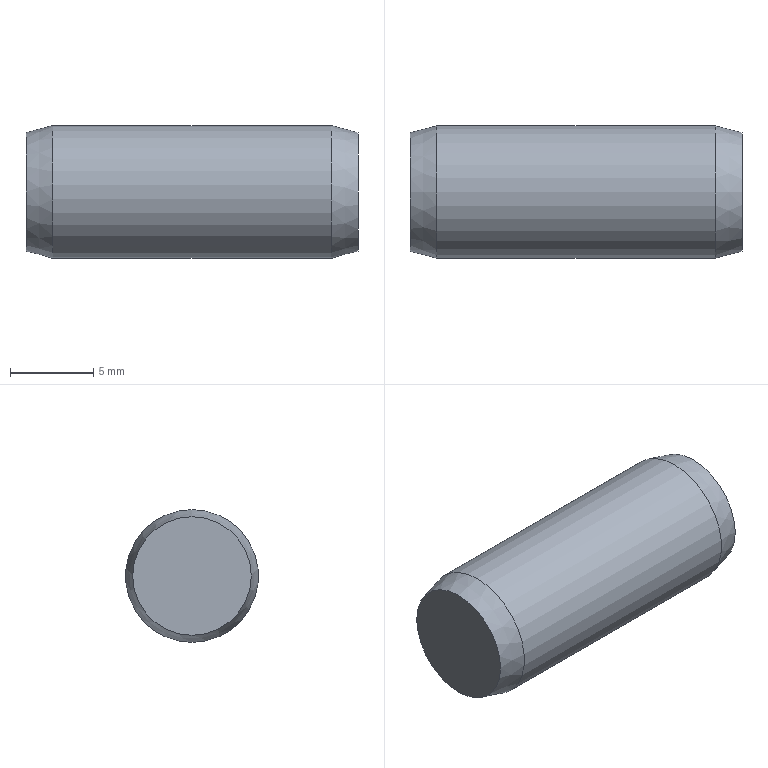Component | NX | GB-T119_1-2000_8X20_2 | 1 solid | 5 faces | box 20 x 8 x 8 mm | volume 989 mm3 | plane 2 | cone 2 | cylinder 1 | commonest cylinder face diameters 8 x1
STEP:
#1=CARTESIAN_POINT('',(0.,0.,0.));
#2=DIRECTION('',(0.,0.,1.));
#3=DIRECTION('',(1.,0.,0.));
#4=AXIS2_PLACEMENT_3D('',#1,#2,#3);
#5=CARTESIAN_POINT('',(-7.89,-28.599,-193.805));
#6=VERTEX_POINT('',#5);
#7=CARTESIAN_POINT('',(-7.89,-28.599,-197.377));
#8=DIRECTION('',(-1.,0.,0.));
#9=DIRECTION('',(0.,0.,1.));
#10=AXIS2_PLACEMENT_3D('',#7,#8,#9);
#11=CIRCLE('',#10,3.571);
#12=CARTESIAN_POINT('',(-7.89,-28.599,-197.377));
#13=DIRECTION('',(-1.,0.,0.));
#14=DIRECTION('',(0.,0.,1.));
#15=AXIS2_PLACEMENT_3D('',#12,#13,#14);
#16=PLANE('',#15);
#17=CARTESIAN_POINT('',(0.,0.));
#18=DIRECTION('',(1.,0.));
#19=AXIS2_PLACEMENT_2D('',#17,#18);
#20=CIRCLE('',#19,3.571);
#21=(GEOMETRIC_REPRESENTATION_CONTEXT(2)PARAMETRIC_REPRESENTATION_CONTEXT()REPRESENTATION_CONTEXT('',''));
#22=DEFINITIONAL_REPRESENTATION('',(#20),#21);
#23=PCURVE('',#16,#22);
#24=CARTESIAN_POINT('',(-7.89,-28.599,-197.377));
#25=DIRECTION('',(1.,0.,0.));
#26=DIRECTION('',(0.,0.,-1.));
#27=AXIS2_PLACEMENT_3D('',#24,#25,#26);
#28=CONICAL_SURFACE('',#27,3.571,0.2618);
#29=CARTESIAN_POINT('',(9.425,-0.));
#30=DIRECTION('',(-1.,0.));
#31=VECTOR('',#30,1.);
#32=LINE('',#29,#31);
#33=(GEOMETRIC_REPRESENTATION_CONTEXT(2)PARAMETRIC_REPRESENTATION_CONTEXT()REPRESENTATION_CONTEXT('',''));
#34=DEFINITIONAL_REPRESENTATION('',(#32),#33);
#35=PCURVE('',#28,#34);
#36=SURFACE_CURVE('',#11,(#23,#35),.PCURVE_S1.);
#37=EDGE_CURVE('',#6,#6,#36,.T.);
#38=ORIENTED_EDGE('',*,*,#37,.T.);
#39=EDGE_LOOP('',(#38));
#40=FACE_BOUND('',#39,.T.);
#41=ADVANCED_FACE('',(#40),#16,.T.);
#42=CARTESIAN_POINT('',(-6.29,-28.599,-193.377));
#43=VERTEX_POINT('',#42);
#44=CARTESIAN_POINT('',(-6.29,-28.599,-197.377));
#45=DIRECTION('',(-1.,0.,0.));
#46=DIRECTION('',(0.,0.,1.));
#47=AXIS2_PLACEMENT_3D('',#44,#45,#46);
#48=CIRCLE('',#47,4.);
#49=CARTESIAN_POINT('',(9.425,1.6));
#50=DIRECTION('',(-1.,0.));
#51=VECTOR('',#50,1.);
#52=LINE('',#49,#51);
#53=(GEOMETRIC_REPRESENTATION_CONTEXT(2)PARAMETRIC_REPRESENTATION_CONTEXT()REPRESENTATION_CONTEXT('',''));
#54=DEFINITIONAL_REPRESENTATION('',(#52),#53);
#55=PCURVE('',#28,#54);
#56=CARTESIAN_POINT('',(12.11,-28.599,-197.377));
#57=DIRECTION('',(-1.,0.,0.));
#58=DIRECTION('',(0.,0.,1.));
#59=AXIS2_PLACEMENT_3D('',#56,#57,#58);
#60=CYLINDRICAL_SURFACE('',#59,4.);
#61=CARTESIAN_POINT('',(0.,18.4));
#62=DIRECTION('',(1.,0.));
#63=VECTOR('',#62,1.);
#64=LINE('',#61,#63);
#65=(GEOMETRIC_REPRESENTATION_CONTEXT(2)PARAMETRIC_REPRESENTATION_CONTEXT()REPRESENTATION_CONTEXT('',''));
#66=DEFINITIONAL_REPRESENTATION('',(#64),#65);
#67=PCURVE('',#60,#66);
#68=SURFACE_CURVE('',#48,(#55,#67),.PCURVE_S1.);
#69=EDGE_CURVE('',#43,#43,#68,.T.);
#70=ORIENTED_EDGE('',*,*,#69,.T.);
#71=CARTESIAN_POINT('',(-7.89,-28.599,-193.805));
#72=CARTESIAN_POINT('',(-6.29,-28.599,-193.377));
#73=B_SPLINE_CURVE_WITH_KNOTS('',1,(#71,#72),.UNSPECIFIED.,.F.,.F.,(2,2),(-0.,1.656),.PIECEWISE_BEZIER_KNOTS.);
#74=CARTESIAN_POINT('',(3.142,0.));
#75=DIRECTION('',(0.,1.));
#76=VECTOR('',#75,1.);
#77=LINE('',#74,#76);
#78=(GEOMETRIC_REPRESENTATION_CONTEXT(2)PARAMETRIC_REPRESENTATION_CONTEXT()REPRESENTATION_CONTEXT('',''));
#79=DEFINITIONAL_REPRESENTATION('',(#77),#78);
#80=PCURVE('',#28,#79);
#81=CARTESIAN_POINT('',(9.425,0.));
#82=DIRECTION('',(0.,1.));
#83=VECTOR('',#82,1.);
#84=LINE('',#81,#83);
#85=(GEOMETRIC_REPRESENTATION_CONTEXT(2)PARAMETRIC_REPRESENTATION_CONTEXT()REPRESENTATION_CONTEXT('',''));
#86=DEFINITIONAL_REPRESENTATION('',(#84),#85);
#87=PCURVE('',#28,#86);
#88=SEAM_CURVE('',#73,(#80,#87),.PCURVE_S1.);
#89=EDGE_CURVE('',#6,#43,#88,.T.);
#90=ORIENTED_EDGE('',*,*,#89,.F.);
#91=ORIENTED_EDGE('',*,*,#37,.F.);
#92=ORIENTED_EDGE('',*,*,#89,.T.);
#93=EDGE_LOOP('',(#70,#90,#91,#92));
#94=FACE_BOUND('',#93,.T.);
#95=ADVANCED_FACE('',(#94),#28,.T.);
#96=CARTESIAN_POINT('',(10.51,-28.599,-193.377));
#97=VERTEX_POINT('',#96);
#98=CARTESIAN_POINT('',(10.51,-28.599,-197.377));
#99=DIRECTION('',(-1.,0.,0.));
#100=DIRECTION('',(0.,0.,1.));
#101=AXIS2_PLACEMENT_3D('',#98,#99,#100);
#102=CIRCLE('',#101,4.);
#103=CARTESIAN_POINT('',(0.,1.6));
#104=DIRECTION('',(1.,0.));
#105=VECTOR('',#104,1.);
#106=LINE('',#103,#105);
#107=(GEOMETRIC_REPRESENTATION_CONTEXT(2)PARAMETRIC_REPRESENTATION_CONTEXT()REPRESENTATION_CONTEXT('',''));
#108=DEFINITIONAL_REPRESENTATION('',(#106),#107);
#109=PCURVE('',#60,#108);
#110=CARTESIAN_POINT('',(10.51,-28.599,-197.377));
#111=DIRECTION('',(-1.,0.,0.));
#112=DIRECTION('',(0.,0.,1.));
#113=AXIS2_PLACEMENT_3D('',#110,#111,#112);
#114=CONICAL_SURFACE('',#113,4.,0.2618);
#115=CARTESIAN_POINT('',(0.,-0.));
#116=DIRECTION('',(1.,0.));
#117=VECTOR('',#116,1.);
#118=LINE('',#115,#117);
#119=(GEOMETRIC_REPRESENTATION_CONTEXT(2)PARAMETRIC_REPRESENTATION_CONTEXT()REPRESENTATION_CONTEXT('',''));
#120=DEFINITIONAL_REPRESENTATION('',(#118),#119);
#121=PCURVE('',#114,#120);
#122=SURFACE_CURVE('',#102,(#109,#121),.PCURVE_S1.);
#123=EDGE_CURVE('',#97,#97,#122,.T.);
#124=ORIENTED_EDGE('',*,*,#123,.T.);
#125=CARTESIAN_POINT('',(10.51,-28.599,-193.377));
#126=CARTESIAN_POINT('',(-6.29,-28.599,-193.377));
#127=B_SPLINE_CURVE_WITH_KNOTS('',1,(#125,#126),.UNSPECIFIED.,.F.,.F.,(2,2),(1.6,18.4),.PIECEWISE_BEZIER_KNOTS.);
#128=CARTESIAN_POINT('',(6.283,0.));
#129=DIRECTION('',(0.,1.));
#130=VECTOR('',#129,1.);
#131=LINE('',#128,#130);
#132=(GEOMETRIC_REPRESENTATION_CONTEXT(2)PARAMETRIC_REPRESENTATION_CONTEXT()REPRESENTATION_CONTEXT('',''));
#133=DEFINITIONAL_REPRESENTATION('',(#131),#132);
#134=PCURVE('',#60,#133);
#135=CARTESIAN_POINT('',(0.,0.));
#136=DIRECTION('',(0.,1.));
#137=VECTOR('',#136,1.);
#138=LINE('',#135,#137);
#139=(GEOMETRIC_REPRESENTATION_CONTEXT(2)PARAMETRIC_REPRESENTATION_CONTEXT()REPRESENTATION_CONTEXT('',''));
#140=DEFINITIONAL_REPRESENTATION('',(#138),#139);
#141=PCURVE('',#60,#140);
#142=SEAM_CURVE('',#127,(#134,#141),.PCURVE_S1.);
#143=EDGE_CURVE('',#97,#43,#142,.T.);
#144=ORIENTED_EDGE('',*,*,#143,.T.);
#145=ORIENTED_EDGE('',*,*,#69,.F.);
#146=ORIENTED_EDGE('',*,*,#143,.F.);
#147=EDGE_LOOP('',(#124,#144,#145,#146));
#148=FACE_BOUND('',#147,.T.);
#149=ADVANCED_FACE('',(#148),#60,.T.);
#150=CARTESIAN_POINT('',(12.11,-28.599,-193.805));
#151=VERTEX_POINT('',#150);
#152=CARTESIAN_POINT('',(12.11,-28.599,-197.377));
#153=DIRECTION('',(-1.,0.,0.));
#154=DIRECTION('',(0.,0.,1.));
#155=AXIS2_PLACEMENT_3D('',#152,#153,#154);
#156=CIRCLE('',#155,3.571);
#157=CARTESIAN_POINT('',(0.,-1.6));
#158=DIRECTION('',(1.,0.));
#159=VECTOR('',#158,1.);
#160=LINE('',#157,#159);
#161=(GEOMETRIC_REPRESENTATION_CONTEXT(2)PARAMETRIC_REPRESENTATION_CONTEXT()REPRESENTATION_CONTEXT('',''));
#162=DEFINITIONAL_REPRESENTATION('',(#160),#161);
#163=PCURVE('',#114,#162);
#164=CARTESIAN_POINT('',(12.11,-28.599,-200.948));
#165=DIRECTION('',(1.,0.,0.));
#166=DIRECTION('',(0.,0.,-1.));
#167=AXIS2_PLACEMENT_3D('',#164,#165,#166);
#168=PLANE('',#167);
#169=CARTESIAN_POINT('',(-7.143,0.));
#170=CARTESIAN_POINT('',(-7.143,6.186));
#171=CARTESIAN_POINT('',(-1.786,3.093));
#172=CARTESIAN_POINT('',(3.571,0.));
#173=CARTESIAN_POINT('',(-1.786,-3.093));
#174=CARTESIAN_POINT('',(-7.143,-6.186));
#175=CARTESIAN_POINT('',(-7.143,0.));
#176=(BOUNDED_CURVE()B_SPLINE_CURVE(2,(#169,#170,#171,#172,#173,#174,#175),.UNSPECIFIED.,.T.,.F.)B_SPLINE_CURVE_WITH_KNOTS((1,2,2,2,2,1),(-2.094,0.,2.094,4.189,6.283,8.378),.UNSPECIFIED.)CURVE()GEOMETRIC_REPRESENTATION_ITEM()RATIONAL_B_SPLINE_CURVE((1.,0.5,1.,0.5,1.,0.5,1.))REPRESENTATION_ITEM(''));
#177=(GEOMETRIC_REPRESENTATION_CONTEXT(2)PARAMETRIC_REPRESENTATION_CONTEXT()REPRESENTATION_CONTEXT('',''));
#178=DEFINITIONAL_REPRESENTATION('',(#176),#177);
#179=PCURVE('',#168,#178);
#180=SURFACE_CURVE('',#156,(#163,#179),.PCURVE_S1.);
#181=EDGE_CURVE('',#151,#151,#180,.T.);
#182=ORIENTED_EDGE('',*,*,#181,.T.);
#183=CARTESIAN_POINT('',(12.11,-28.599,-193.805));
#184=CARTESIAN_POINT('',(10.51,-28.599,-193.377));
#185=B_SPLINE_CURVE_WITH_KNOTS('',1,(#183,#184),.UNSPECIFIED.,.F.,.F.,(2,2),(-1.656,-0.),.PIECEWISE_BEZIER_KNOTS.);
#186=CARTESIAN_POINT('',(6.283,0.));
#187=DIRECTION('',(0.,1.));
#188=VECTOR('',#187,1.);
#189=LINE('',#186,#188);
#190=(GEOMETRIC_REPRESENTATION_CONTEXT(2)PARAMETRIC_REPRESENTATION_CONTEXT()REPRESENTATION_CONTEXT('',''));
#191=DEFINITIONAL_REPRESENTATION('',(#189),#190);
#192=PCURVE('',#114,#191);
#193=CARTESIAN_POINT('',(0.,0.));
#194=DIRECTION('',(0.,1.));
#195=VECTOR('',#194,1.);
#196=LINE('',#193,#195);
#197=(GEOMETRIC_REPRESENTATION_CONTEXT(2)PARAMETRIC_REPRESENTATION_CONTEXT()REPRESENTATION_CONTEXT('',''));
#198=DEFINITIONAL_REPRESENTATION('',(#196),#197);
#199=PCURVE('',#114,#198);
#200=SEAM_CURVE('',#185,(#192,#199),.PCURVE_S1.);
#201=EDGE_CURVE('',#151,#97,#200,.T.);
#202=ORIENTED_EDGE('',*,*,#201,.T.);
#203=ORIENTED_EDGE('',*,*,#123,.F.);
#204=ORIENTED_EDGE('',*,*,#201,.F.);
#205=EDGE_LOOP('',(#182,#202,#203,#204));
#206=FACE_BOUND('',#205,.T.);
#207=ADVANCED_FACE('',(#206),#114,.T.);
#208=ORIENTED_EDGE('',*,*,#181,.F.);
#209=EDGE_LOOP('',(#208));
#210=FACE_BOUND('',#209,.T.);
#211=ADVANCED_FACE('',(#210),#168,.T.);
#212=CLOSED_SHELL('',(#41,#95,#149,#207,#211));
#213=MANIFOLD_SOLID_BREP('',#212);
#214=(LENGTH_UNIT()NAMED_UNIT(*)SI_UNIT(.MILLI.,.METRE.));
#215=UNCERTAINTY_MEASURE_WITH_UNIT(LENGTH_MEASURE(0.00001),#214,'','');
#216=(NAMED_UNIT(*)PLANE_ANGLE_UNIT()SI_UNIT($,.RADIAN.));
#217=(NAMED_UNIT(*)SI_UNIT($,.STERADIAN.)SOLID_ANGLE_UNIT());
#218=(GEOMETRIC_REPRESENTATION_CONTEXT(3)GLOBAL_UNCERTAINTY_ASSIGNED_CONTEXT((#215))GLOBAL_UNIT_ASSIGNED_CONTEXT((#214,#216,#217))REPRESENTATION_CONTEXT('',''));
#219=ADVANCED_BREP_SHAPE_REPRESENTATION('',(#4,#213),#218);